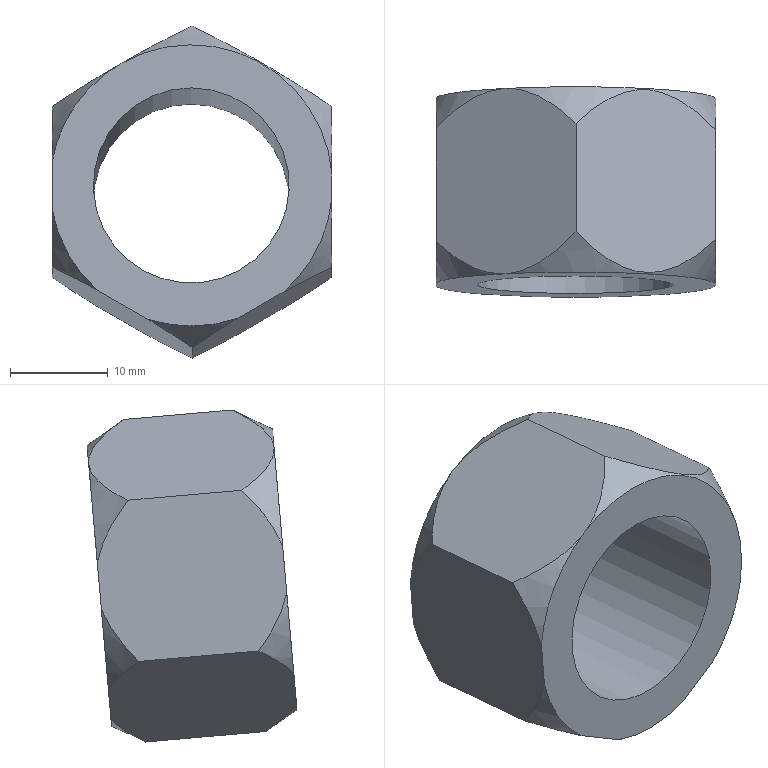Component | NX | NUT | 1 solid | 19 faces | volume 7342 mm3 | cone 10 | plane 8 | cylinder 1 | commonest cylinder face diameters 20 x1